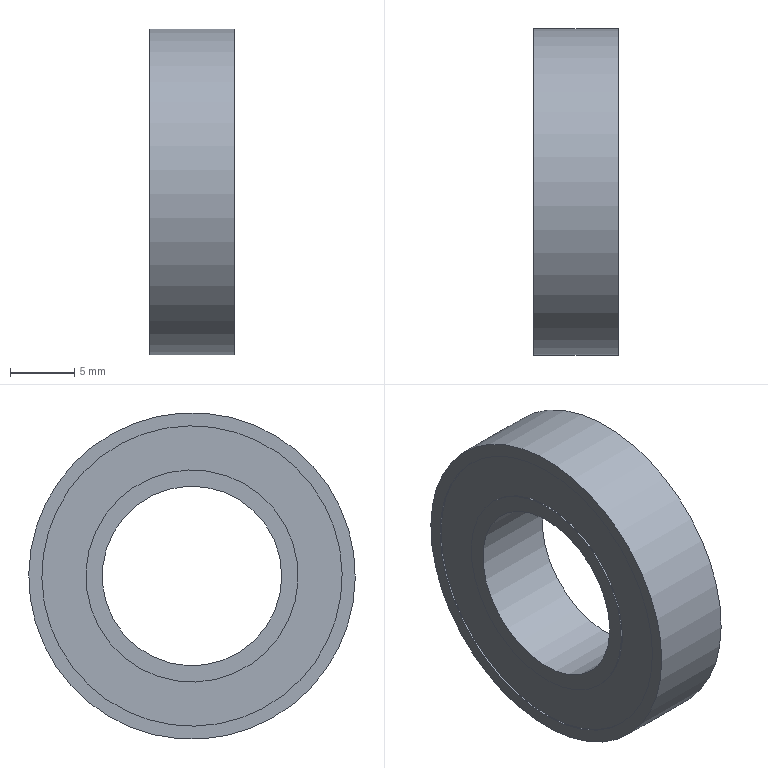Component | NX | BEARINGBIG | 3 solids | 12 faces | box 6.54 x 25.4 x 25.4 mm | volume 2257 mm3 | cylinder 6 | plane 6 | commonest cylinder face diameters 23.368 x2 16.51 x2 25.4 x1 13.97 x1
STEP:
#1=CARTESIAN_POINT('',(0.,0.,0.));
#2=DIRECTION('',(0.,0.,1.));
#3=DIRECTION('',(1.,0.,0.));
#4=AXIS2_PLACEMENT_3D('',#1,#2,#3);
#5=CARTESIAN_POINT('',(6.54,-10.403,-7.284));
#6=VERTEX_POINT('',#5);
#7=CARTESIAN_POINT('',(6.54,0.,0.));
#8=DIRECTION('',(1.,0.,0.));
#9=DIRECTION('',(0.,-0.8192,-0.5736));
#10=AXIS2_PLACEMENT_3D('',#7,#8,#9);
#11=CIRCLE('',#10,12.7);
#12=CARTESIAN_POINT('',(6.54,0.,0.));
#13=DIRECTION('',(-1.,0.,0.));
#14=DIRECTION('',(0.,0.5736,-0.8192));
#15=AXIS2_PLACEMENT_3D('',#12,#13,#14);
#16=CYLINDRICAL_SURFACE('',#15,12.7);
#17=CARTESIAN_POINT('',(7.854,0.));
#18=DIRECTION('',(-1.,0.));
#19=VECTOR('',#18,1.);
#20=LINE('',#17,#19);
#21=(GEOMETRIC_REPRESENTATION_CONTEXT(2)PARAMETRIC_REPRESENTATION_CONTEXT()REPRESENTATION_CONTEXT('',''));
#22=DEFINITIONAL_REPRESENTATION('',(#20),#21);
#23=PCURVE('',#16,#22);
#24=CARTESIAN_POINT('',(6.54,0.,0.));
#25=DIRECTION('',(1.,0.,0.));
#26=DIRECTION('',(0.,-0.5736,0.8192));
#27=AXIS2_PLACEMENT_3D('',#24,#25,#26);
#28=PLANE('',#27);
#29=CARTESIAN_POINT('',(0.,0.));
#30=DIRECTION('',(0.,1.));
#31=AXIS2_PLACEMENT_2D('',#29,#30);
#32=CIRCLE('',#31,12.7);
#33=(GEOMETRIC_REPRESENTATION_CONTEXT(2)PARAMETRIC_REPRESENTATION_CONTEXT()REPRESENTATION_CONTEXT('',''));
#34=DEFINITIONAL_REPRESENTATION('',(#32),#33);
#35=PCURVE('',#28,#34);
#36=SURFACE_CURVE('',#11,(#23,#35),.PCURVE_S1.);
#37=EDGE_CURVE('',#6,#6,#36,.T.);
#38=ORIENTED_EDGE('',*,*,#37,.F.);
#39=CARTESIAN_POINT('',(0.,-10.403,-7.284));
#40=VERTEX_POINT('',#39);
#41=CARTESIAN_POINT('',(6.54,-10.403,-7.284));
#42=CARTESIAN_POINT('',(0.,-10.403,-7.284));
#43=B_SPLINE_CURVE_WITH_KNOTS('',1,(#41,#42),.UNSPECIFIED.,.F.,.F.,(2,2),(0.,6.54),.PIECEWISE_BEZIER_KNOTS.);
#44=CARTESIAN_POINT('',(7.854,0.));
#45=DIRECTION('',(0.,1.));
#46=VECTOR('',#45,1.);
#47=LINE('',#44,#46);
#48=(GEOMETRIC_REPRESENTATION_CONTEXT(2)PARAMETRIC_REPRESENTATION_CONTEXT()REPRESENTATION_CONTEXT('',''));
#49=DEFINITIONAL_REPRESENTATION('',(#47),#48);
#50=PCURVE('',#16,#49);
#51=CARTESIAN_POINT('',(1.571,0.));
#52=DIRECTION('',(0.,1.));
#53=VECTOR('',#52,1.);
#54=LINE('',#51,#53);
#55=(GEOMETRIC_REPRESENTATION_CONTEXT(2)PARAMETRIC_REPRESENTATION_CONTEXT()REPRESENTATION_CONTEXT('',''));
#56=DEFINITIONAL_REPRESENTATION('',(#54),#55);
#57=PCURVE('',#16,#56);
#58=SEAM_CURVE('',#43,(#50,#57),.PCURVE_S1.);
#59=EDGE_CURVE('',#6,#40,#58,.T.);
#60=ORIENTED_EDGE('',*,*,#59,.T.);
#61=CARTESIAN_POINT('',(0.,0.,0.));
#62=DIRECTION('',(1.,0.,0.));
#63=DIRECTION('',(0.,-0.8192,-0.5736));
#64=AXIS2_PLACEMENT_3D('',#61,#62,#63);
#65=CIRCLE('',#64,12.7);
#66=CARTESIAN_POINT('',(7.854,6.54));
#67=DIRECTION('',(-1.,0.));
#68=VECTOR('',#67,1.);
#69=LINE('',#66,#68);
#70=(GEOMETRIC_REPRESENTATION_CONTEXT(2)PARAMETRIC_REPRESENTATION_CONTEXT()REPRESENTATION_CONTEXT('',''));
#71=DEFINITIONAL_REPRESENTATION('',(#69),#70);
#72=PCURVE('',#16,#71);
#73=CARTESIAN_POINT('',(0.,0.,0.));
#74=DIRECTION('',(1.,0.,0.));
#75=DIRECTION('',(0.,-0.5736,0.8192));
#76=AXIS2_PLACEMENT_3D('',#73,#74,#75);
#77=PLANE('',#76);
#78=CARTESIAN_POINT('',(0.,0.));
#79=DIRECTION('',(0.,1.));
#80=AXIS2_PLACEMENT_2D('',#78,#79);
#81=CIRCLE('',#80,12.7);
#82=(GEOMETRIC_REPRESENTATION_CONTEXT(2)PARAMETRIC_REPRESENTATION_CONTEXT()REPRESENTATION_CONTEXT('',''));
#83=DEFINITIONAL_REPRESENTATION('',(#81),#82);
#84=PCURVE('',#77,#83);
#85=SURFACE_CURVE('',#65,(#72,#84),.PCURVE_S1.);
#86=EDGE_CURVE('',#40,#40,#85,.T.);
#87=ORIENTED_EDGE('',*,*,#86,.T.);
#88=ORIENTED_EDGE('',*,*,#59,.F.);
#89=EDGE_LOOP('',(#38,#60,#87,#88));
#90=FACE_BOUND('',#89,.T.);
#91=ADVANCED_FACE('',(#90),#16,.T.);
#92=CARTESIAN_POINT('',(6.54,-9.571,-6.702));
#93=VERTEX_POINT('',#92);
#94=CARTESIAN_POINT('',(6.54,0.,0.));
#95=DIRECTION('',(-1.,0.,0.));
#96=DIRECTION('',(0.,-0.8192,-0.5736));
#97=AXIS2_PLACEMENT_3D('',#94,#95,#96);
#98=CIRCLE('',#97,11.684);
#99=CARTESIAN_POINT('',(6.54,0.,0.));
#100=DIRECTION('',(-1.,0.,0.));
#101=DIRECTION('',(0.,0.5736,-0.8192));
#102=AXIS2_PLACEMENT_3D('',#99,#100,#101);
#103=CYLINDRICAL_SURFACE('',#102,11.684);
#104=CARTESIAN_POINT('',(1.571,0.));
#105=DIRECTION('',(1.,0.));
#106=VECTOR('',#105,1.);
#107=LINE('',#104,#106);
#108=(GEOMETRIC_REPRESENTATION_CONTEXT(2)PARAMETRIC_REPRESENTATION_CONTEXT()REPRESENTATION_CONTEXT('',''));
#109=DEFINITIONAL_REPRESENTATION('',(#107),#108);
#110=PCURVE('',#103,#109);
#111=CARTESIAN_POINT('',(0.,11.684));
#112=CARTESIAN_POINT('',(20.237,11.684));
#113=CARTESIAN_POINT('',(10.119,-5.842));
#114=CARTESIAN_POINT('',(0.,-23.368));
#115=CARTESIAN_POINT('',(-10.119,-5.842));
#116=CARTESIAN_POINT('',(-20.237,11.684));
#117=CARTESIAN_POINT('',(0.,11.684));
#118=(BOUNDED_CURVE()B_SPLINE_CURVE(2,(#111,#112,#113,#114,#115,#116,#117),.UNSPECIFIED.,.T.,.F.)B_SPLINE_CURVE_WITH_KNOTS((1,2,2,2,2,1),(-2.094,0.,2.094,4.189,6.283,8.378),.UNSPECIFIED.)CURVE()GEOMETRIC_REPRESENTATION_ITEM()RATIONAL_B_SPLINE_CURVE((1.,0.5,1.,0.5,1.,0.5,1.))REPRESENTATION_ITEM(''));
#119=(GEOMETRIC_REPRESENTATION_CONTEXT(2)PARAMETRIC_REPRESENTATION_CONTEXT()REPRESENTATION_CONTEXT('',''));
#120=DEFINITIONAL_REPRESENTATION('',(#118),#119);
#121=PCURVE('',#28,#120);
#122=SURFACE_CURVE('',#98,(#110,#121),.PCURVE_S1.);
#123=EDGE_CURVE('',#93,#93,#122,.T.);
#124=ORIENTED_EDGE('',*,*,#123,.T.);
#125=CARTESIAN_POINT('',(0.,-9.571,-6.702));
#126=VERTEX_POINT('',#125);
#127=CARTESIAN_POINT('',(6.54,-9.571,-6.702));
#128=CARTESIAN_POINT('',(0.,-9.571,-6.702));
#129=B_SPLINE_CURVE_WITH_KNOTS('',1,(#127,#128),.UNSPECIFIED.,.F.,.F.,(2,2),(0.,6.54),.PIECEWISE_BEZIER_KNOTS.);
#130=CARTESIAN_POINT('',(7.854,0.));
#131=DIRECTION('',(0.,1.));
#132=VECTOR('',#131,1.);
#133=LINE('',#130,#132);
#134=(GEOMETRIC_REPRESENTATION_CONTEXT(2)PARAMETRIC_REPRESENTATION_CONTEXT()REPRESENTATION_CONTEXT('',''));
#135=DEFINITIONAL_REPRESENTATION('',(#133),#134);
#136=PCURVE('',#103,#135);
#137=CARTESIAN_POINT('',(1.571,0.));
#138=DIRECTION('',(0.,1.));
#139=VECTOR('',#138,1.);
#140=LINE('',#137,#139);
#141=(GEOMETRIC_REPRESENTATION_CONTEXT(2)PARAMETRIC_REPRESENTATION_CONTEXT()REPRESENTATION_CONTEXT('',''));
#142=DEFINITIONAL_REPRESENTATION('',(#140),#141);
#143=PCURVE('',#103,#142);
#144=SEAM_CURVE('',#129,(#136,#143),.PCURVE_S1.);
#145=EDGE_CURVE('',#93,#126,#144,.T.);
#146=ORIENTED_EDGE('',*,*,#145,.T.);
#147=CARTESIAN_POINT('',(0.,0.,0.));
#148=DIRECTION('',(-1.,0.,0.));
#149=DIRECTION('',(0.,-0.8192,-0.5736));
#150=AXIS2_PLACEMENT_3D('',#147,#148,#149);
#151=CIRCLE('',#150,11.684);
#152=CARTESIAN_POINT('',(1.571,6.54));
#153=DIRECTION('',(1.,0.));
#154=VECTOR('',#153,1.);
#155=LINE('',#152,#154);
#156=(GEOMETRIC_REPRESENTATION_CONTEXT(2)PARAMETRIC_REPRESENTATION_CONTEXT()REPRESENTATION_CONTEXT('',''));
#157=DEFINITIONAL_REPRESENTATION('',(#155),#156);
#158=PCURVE('',#103,#157);
#159=CARTESIAN_POINT('',(0.,11.684));
#160=CARTESIAN_POINT('',(20.237,11.684));
#161=CARTESIAN_POINT('',(10.119,-5.842));
#162=CARTESIAN_POINT('',(0.,-23.368));
#163=CARTESIAN_POINT('',(-10.119,-5.842));
#164=CARTESIAN_POINT('',(-20.237,11.684));
#165=CARTESIAN_POINT('',(0.,11.684));
#166=(BOUNDED_CURVE()B_SPLINE_CURVE(2,(#159,#160,#161,#162,#163,#164,#165),.UNSPECIFIED.,.T.,.F.)B_SPLINE_CURVE_WITH_KNOTS((1,2,2,2,2,1),(-2.094,0.,2.094,4.189,6.283,8.378),.UNSPECIFIED.)CURVE()GEOMETRIC_REPRESENTATION_ITEM()RATIONAL_B_SPLINE_CURVE((1.,0.5,1.,0.5,1.,0.5,1.))REPRESENTATION_ITEM(''));
#167=(GEOMETRIC_REPRESENTATION_CONTEXT(2)PARAMETRIC_REPRESENTATION_CONTEXT()REPRESENTATION_CONTEXT('',''));
#168=DEFINITIONAL_REPRESENTATION('',(#166),#167);
#169=PCURVE('',#77,#168);
#170=SURFACE_CURVE('',#151,(#158,#169),.PCURVE_S1.);
#171=EDGE_CURVE('',#126,#126,#170,.T.);
#172=ORIENTED_EDGE('',*,*,#171,.F.);
#173=ORIENTED_EDGE('',*,*,#145,.F.);
#174=EDGE_LOOP('',(#124,#146,#172,#173));
#175=FACE_BOUND('',#174,.F.);
#176=ADVANCED_FACE('',(#175),#103,.F.);
#177=ORIENTED_EDGE('',*,*,#37,.T.);
#178=EDGE_LOOP('',(#177));
#179=FACE_BOUND('',#178,.T.);
#180=ORIENTED_EDGE('',*,*,#123,.T.);
#181=EDGE_LOOP('',(#180));
#182=FACE_BOUND('',#181,.T.);
#183=ADVANCED_FACE('',(#179,#182),#28,.T.);
#184=ORIENTED_EDGE('',*,*,#86,.F.);
#185=EDGE_LOOP('',(#184));
#186=FACE_BOUND('',#185,.T.);
#187=ORIENTED_EDGE('',*,*,#171,.F.);
#188=EDGE_LOOP('',(#187));
#189=FACE_BOUND('',#188,.T.);
#190=ADVANCED_FACE('',(#186,#189),#77,.F.);
#191=CLOSED_SHELL('',(#91,#176,#183,#190));
#192=MANIFOLD_SOLID_BREP('',#191);
#193=(LENGTH_UNIT()NAMED_UNIT(*)SI_UNIT(.MILLI.,.METRE.));
#194=UNCERTAINTY_MEASURE_WITH_UNIT(LENGTH_MEASURE(0.00001),#193,'','');
#195=(NAMED_UNIT(*)PLANE_ANGLE_UNIT()SI_UNIT($,.RADIAN.));
#196=(NAMED_UNIT(*)SI_UNIT($,.STERADIAN.)SOLID_ANGLE_UNIT());
#197=(GEOMETRIC_REPRESENTATION_CONTEXT(3)GLOBAL_UNCERTAINTY_ASSIGNED_CONTEXT((#194))GLOBAL_UNIT_ASSIGNED_CONTEXT((#193,#195,#196))REPRESENTATION_CONTEXT('',''));
#198=ADVANCED_BREP_SHAPE_REPRESENTATION('',(#4,#192),#197);
#199=CARTESIAN_POINT('',(0.,0.,0.));
#200=DIRECTION('',(0.,0.,1.));
#201=DIRECTION('',(1.,0.,0.));
#202=AXIS2_PLACEMENT_3D('',#199,#200,#201);
#203=CARTESIAN_POINT('',(0.,0.,0.));
#204=DIRECTION('',(0.,0.,1.));
#205=DIRECTION('',(1.,0.,0.));
#206=AXIS2_PLACEMENT_3D('',#203,#204,#205);
#207=CARTESIAN_POINT('',(0.,0.,0.));
#208=DIRECTION('',(0.,0.,1.));
#209=DIRECTION('',(1.,0.,0.));
#210=AXIS2_PLACEMENT_3D('',#207,#208,#209);
#211=(LENGTH_UNIT()NAMED_UNIT(*)SI_UNIT(.MILLI.,.METRE.));
#212=UNCERTAINTY_MEASURE_WITH_UNIT(LENGTH_MEASURE(0.00001),#211,'','');
#213=(NAMED_UNIT(*)PLANE_ANGLE_UNIT()SI_UNIT($,.RADIAN.));
#214=(NAMED_UNIT(*)SI_UNIT($,.STERADIAN.)SOLID_ANGLE_UNIT());
#215=(GEOMETRIC_REPRESENTATION_CONTEXT(3)GLOBAL_UNCERTAINTY_ASSIGNED_CONTEXT((#212))GLOBAL_UNIT_ASSIGNED_CONTEXT((#211,#213,#214))REPRESENTATION_CONTEXT('',''));
#216=SHAPE_REPRESENTATION('',(#4,#202,#206,#210),#215);
#217=ITEM_DEFINED_TRANSFORMATION('','',#4,#202);
#218=(REPRESENTATION_RELATIONSHIP('','',#198,#216)REPRESENTATION_RELATIONSHIP_WITH_TRANSFORMATION(#217)SHAPE_REPRESENTATION_RELATIONSHIP());
#219=CARTESIAN_POINT('',(6.54,-6.762,-4.735));
#220=VERTEX_POINT('',#219);
#221=CARTESIAN_POINT('',(6.54,0.,0.));
#222=DIRECTION('',(-1.,0.,0.));
#223=DIRECTION('',(0.,-0.8192,-0.5736));
#224=AXIS2_PLACEMENT_3D('',#221,#222,#223);
#225=CIRCLE('',#224,8.255);
#226=CARTESIAN_POINT('',(6.54,0.,0.));
#227=DIRECTION('',(-1.,0.,0.));
#228=DIRECTION('',(0.,0.5736,-0.8192));
#229=AXIS2_PLACEMENT_3D('',#226,#227,#228);
#230=CYLINDRICAL_SURFACE('',#229,8.255);
#231=CARTESIAN_POINT('',(1.571,0.));
#232=DIRECTION('',(1.,0.));
#233=VECTOR('',#232,1.);
#234=LINE('',#231,#233);
#235=(GEOMETRIC_REPRESENTATION_CONTEXT(2)PARAMETRIC_REPRESENTATION_CONTEXT()REPRESENTATION_CONTEXT('',''));
#236=DEFINITIONAL_REPRESENTATION('',(#234),#235);
#237=PCURVE('',#230,#236);
#238=CARTESIAN_POINT('',(6.54,0.,0.));
#239=DIRECTION('',(1.,0.,0.));
#240=DIRECTION('',(0.,-0.5736,0.8192));
#241=AXIS2_PLACEMENT_3D('',#238,#239,#240);
#242=PLANE('',#241);
#243=CARTESIAN_POINT('',(0.,8.255));
#244=CARTESIAN_POINT('',(14.298,8.255));
#245=CARTESIAN_POINT('',(7.149,-4.128));
#246=CARTESIAN_POINT('',(0.,-16.51));
#247=CARTESIAN_POINT('',(-7.149,-4.128));
#248=CARTESIAN_POINT('',(-14.298,8.255));
#249=CARTESIAN_POINT('',(0.,8.255));
#250=(BOUNDED_CURVE()B_SPLINE_CURVE(2,(#243,#244,#245,#246,#247,#248,#249),.UNSPECIFIED.,.T.,.F.)B_SPLINE_CURVE_WITH_KNOTS((1,2,2,2,2,1),(-2.094,0.,2.094,4.189,6.283,8.378),.UNSPECIFIED.)CURVE()GEOMETRIC_REPRESENTATION_ITEM()RATIONAL_B_SPLINE_CURVE((1.,0.5,1.,0.5,1.,0.5,1.))REPRESENTATION_ITEM(''));
#251=(GEOMETRIC_REPRESENTATION_CONTEXT(2)PARAMETRIC_REPRESENTATION_CONTEXT()REPRESENTATION_CONTEXT('',''));
#252=DEFINITIONAL_REPRESENTATION('',(#250),#251);
#253=PCURVE('',#242,#252);
#254=SURFACE_CURVE('',#225,(#237,#253),.PCURVE_S1.);
#255=EDGE_CURVE('',#220,#220,#254,.T.);
#256=ORIENTED_EDGE('',*,*,#255,.T.);
#257=CARTESIAN_POINT('',(0.,-6.762,-4.735));
#258=VERTEX_POINT('',#257);
#259=CARTESIAN_POINT('',(6.54,-6.762,-4.735));
#260=CARTESIAN_POINT('',(0.,-6.762,-4.735));
#261=B_SPLINE_CURVE_WITH_KNOTS('',1,(#259,#260),.UNSPECIFIED.,.F.,.F.,(2,2),(0.,6.54),.PIECEWISE_BEZIER_KNOTS.);
#262=CARTESIAN_POINT('',(7.854,0.));
#263=DIRECTION('',(0.,1.));
#264=VECTOR('',#263,1.);
#265=LINE('',#262,#264);
#266=(GEOMETRIC_REPRESENTATION_CONTEXT(2)PARAMETRIC_REPRESENTATION_CONTEXT()REPRESENTATION_CONTEXT('',''));
#267=DEFINITIONAL_REPRESENTATION('',(#265),#266);
#268=PCURVE('',#230,#267);
#269=CARTESIAN_POINT('',(1.571,0.));
#270=DIRECTION('',(0.,1.));
#271=VECTOR('',#270,1.);
#272=LINE('',#269,#271);
#273=(GEOMETRIC_REPRESENTATION_CONTEXT(2)PARAMETRIC_REPRESENTATION_CONTEXT()REPRESENTATION_CONTEXT('',''));
#274=DEFINITIONAL_REPRESENTATION('',(#272),#273);
#275=PCURVE('',#230,#274);
#276=SEAM_CURVE('',#261,(#268,#275),.PCURVE_S1.);
#277=EDGE_CURVE('',#220,#258,#276,.T.);
#278=ORIENTED_EDGE('',*,*,#277,.T.);
#279=CARTESIAN_POINT('',(0.,0.,0.));
#280=DIRECTION('',(-1.,0.,0.));
#281=DIRECTION('',(0.,-0.8192,-0.5736));
#282=AXIS2_PLACEMENT_3D('',#279,#280,#281);
#283=CIRCLE('',#282,8.255);
#284=CARTESIAN_POINT('',(1.571,6.54));
#285=DIRECTION('',(1.,0.));
#286=VECTOR('',#285,1.);
#287=LINE('',#284,#286);
#288=(GEOMETRIC_REPRESENTATION_CONTEXT(2)PARAMETRIC_REPRESENTATION_CONTEXT()REPRESENTATION_CONTEXT('',''));
#289=DEFINITIONAL_REPRESENTATION('',(#287),#288);
#290=PCURVE('',#230,#289);
#291=CARTESIAN_POINT('',(0.,0.,0.));
#292=DIRECTION('',(1.,0.,0.));
#293=DIRECTION('',(0.,-0.5736,0.8192));
#294=AXIS2_PLACEMENT_3D('',#291,#292,#293);
#295=PLANE('',#294);
#296=CARTESIAN_POINT('',(0.,8.255));
#297=CARTESIAN_POINT('',(14.298,8.255));
#298=CARTESIAN_POINT('',(7.149,-4.128));
#299=CARTESIAN_POINT('',(0.,-16.51));
#300=CARTESIAN_POINT('',(-7.149,-4.128));
#301=CARTESIAN_POINT('',(-14.298,8.255));
#302=CARTESIAN_POINT('',(0.,8.255));
#303=(BOUNDED_CURVE()B_SPLINE_CURVE(2,(#296,#297,#298,#299,#300,#301,#302),.UNSPECIFIED.,.T.,.F.)B_SPLINE_CURVE_WITH_KNOTS((1,2,2,2,2,1),(-2.094,0.,2.094,4.189,6.283,8.378),.UNSPECIFIED.)CURVE()GEOMETRIC_REPRESENTATION_ITEM()RATIONAL_B_SPLINE_CURVE((1.,0.5,1.,0.5,1.,0.5,1.))REPRESENTATION_ITEM(''));
#304=(GEOMETRIC_REPRESENTATION_CONTEXT(2)PARAMETRIC_REPRESENTATION_CONTEXT()REPRESENTATION_CONTEXT('',''));
#305=DEFINITIONAL_REPRESENTATION('',(#303),#304);
#306=PCURVE('',#295,#305);
#307=SURFACE_CURVE('',#283,(#290,#306),.PCURVE_S1.);
#308=EDGE_CURVE('',#258,#258,#307,.T.);
#309=ORIENTED_EDGE('',*,*,#308,.F.);
#310=ORIENTED_EDGE('',*,*,#277,.F.);
#311=EDGE_LOOP('',(#256,#278,#309,#310));
#312=FACE_BOUND('',#311,.T.);
#313=ADVANCED_FACE('',(#312),#230,.T.);
#314=CARTESIAN_POINT('',(6.54,-5.722,-4.006));
#315=VERTEX_POINT('',#314);
#316=CARTESIAN_POINT('',(6.54,0.,0.));
#317=DIRECTION('',(1.,0.,0.));
#318=DIRECTION('',(0.,-0.8192,-0.5736));
#319=AXIS2_PLACEMENT_3D('',#316,#317,#318);
#320=CIRCLE('',#319,6.985);
#321=CARTESIAN_POINT('',(6.54,0.,0.));
#322=DIRECTION('',(-1.,0.,0.));
#323=DIRECTION('',(0.,0.5736,-0.8192));
#324=AXIS2_PLACEMENT_3D('',#321,#322,#323);
#325=CYLINDRICAL_SURFACE('',#324,6.985);
#326=CARTESIAN_POINT('',(7.854,0.));
#327=DIRECTION('',(-1.,0.));
#328=VECTOR('',#327,1.);
#329=LINE('',#326,#328);
#330=(GEOMETRIC_REPRESENTATION_CONTEXT(2)PARAMETRIC_REPRESENTATION_CONTEXT()REPRESENTATION_CONTEXT('',''));
#331=DEFINITIONAL_REPRESENTATION('',(#329),#330);
#332=PCURVE('',#325,#331);
#333=CARTESIAN_POINT('',(0.,0.));
#334=DIRECTION('',(0.,1.));
#335=AXIS2_PLACEMENT_2D('',#333,#334);
#336=CIRCLE('',#335,6.985);
#337=(GEOMETRIC_REPRESENTATION_CONTEXT(2)PARAMETRIC_REPRESENTATION_CONTEXT()REPRESENTATION_CONTEXT('',''));
#338=DEFINITIONAL_REPRESENTATION('',(#336),#337);
#339=PCURVE('',#242,#338);
#340=SURFACE_CURVE('',#320,(#332,#339),.PCURVE_S1.);
#341=EDGE_CURVE('',#315,#315,#340,.T.);
#342=ORIENTED_EDGE('',*,*,#341,.F.);
#343=CARTESIAN_POINT('',(0.,-5.722,-4.006));
#344=VERTEX_POINT('',#343);
#345=CARTESIAN_POINT('',(6.54,-5.722,-4.006));
#346=CARTESIAN_POINT('',(0.,-5.722,-4.006));
#347=B_SPLINE_CURVE_WITH_KNOTS('',1,(#345,#346),.UNSPECIFIED.,.F.,.F.,(2,2),(0.,6.54),.PIECEWISE_BEZIER_KNOTS.);
#348=CARTESIAN_POINT('',(7.854,0.));
#349=DIRECTION('',(0.,1.));
#350=VECTOR('',#349,1.);
#351=LINE('',#348,#350);
#352=(GEOMETRIC_REPRESENTATION_CONTEXT(2)PARAMETRIC_REPRESENTATION_CONTEXT()REPRESENTATION_CONTEXT('',''));
#353=DEFINITIONAL_REPRESENTATION('',(#351),#352);
#354=PCURVE('',#325,#353);
#355=CARTESIAN_POINT('',(1.571,0.));
#356=DIRECTION('',(0.,1.));
#357=VECTOR('',#356,1.);
#358=LINE('',#355,#357);
#359=(GEOMETRIC_REPRESENTATION_CONTEXT(2)PARAMETRIC_REPRESENTATION_CONTEXT()REPRESENTATION_CONTEXT('',''));
#360=DEFINITIONAL_REPRESENTATION('',(#358),#359);
#361=PCURVE('',#325,#360);
#362=SEAM_CURVE('',#347,(#354,#361),.PCURVE_S1.);
#363=EDGE_CURVE('',#315,#344,#362,.T.);
#364=ORIENTED_EDGE('',*,*,#363,.T.);
#365=CARTESIAN_POINT('',(0.,0.,0.));
#366=DIRECTION('',(1.,0.,0.));
#367=DIRECTION('',(0.,-0.8192,-0.5736));
#368=AXIS2_PLACEMENT_3D('',#365,#366,#367);
#369=CIRCLE('',#368,6.985);
#370=CARTESIAN_POINT('',(7.854,6.54));
#371=DIRECTION('',(-1.,0.));
#372=VECTOR('',#371,1.);
#373=LINE('',#370,#372);
#374=(GEOMETRIC_REPRESENTATION_CONTEXT(2)PARAMETRIC_REPRESENTATION_CONTEXT()REPRESENTATION_CONTEXT('',''));
#375=DEFINITIONAL_REPRESENTATION('',(#373),#374);
#376=PCURVE('',#325,#375);
#377=CARTESIAN_POINT('',(0.,0.));
#378=DIRECTION('',(0.,1.));
#379=AXIS2_PLACEMENT_2D('',#377,#378);
#380=CIRCLE('',#379,6.985);
#381=(GEOMETRIC_REPRESENTATION_CONTEXT(2)PARAMETRIC_REPRESENTATION_CONTEXT()REPRESENTATION_CONTEXT('',''));
#382=DEFINITIONAL_REPRESENTATION('',(#380),#381);
#383=PCURVE('',#295,#382);
#384=SURFACE_CURVE('',#369,(#376,#383),.PCURVE_S1.);
#385=EDGE_CURVE('',#344,#344,#384,.T.);
#386=ORIENTED_EDGE('',*,*,#385,.T.);
#387=ORIENTED_EDGE('',*,*,#363,.F.);
#388=EDGE_LOOP('',(#342,#364,#386,#387));
#389=FACE_BOUND('',#388,.F.);
#390=ADVANCED_FACE('',(#389),#325,.F.);
#391=ORIENTED_EDGE('',*,*,#255,.F.);
#392=EDGE_LOOP('',(#391));
#393=FACE_BOUND('',#392,.T.);
#394=ORIENTED_EDGE('',*,*,#341,.F.);
#395=EDGE_LOOP('',(#394));
#396=FACE_BOUND('',#395,.T.);
#397=ADVANCED_FACE('',(#393,#396),#242,.T.);
#398=ORIENTED_EDGE('',*,*,#308,.T.);
#399=EDGE_LOOP('',(#398));
#400=FACE_BOUND('',#399,.T.);
#401=ORIENTED_EDGE('',*,*,#385,.T.);
#402=EDGE_LOOP('',(#401));
#403=FACE_BOUND('',#402,.T.);
#404=ADVANCED_FACE('',(#400,#403),#295,.F.);
#405=CLOSED_SHELL('',(#313,#390,#397,#404));
#406=MANIFOLD_SOLID_BREP('',#405);
#407=(LENGTH_UNIT()NAMED_UNIT(*)SI_UNIT(.MILLI.,.METRE.));
#408=UNCERTAINTY_MEASURE_WITH_UNIT(LENGTH_MEASURE(0.00001),#407,'','');
#409=(NAMED_UNIT(*)PLANE_ANGLE_UNIT()SI_UNIT($,.RADIAN.));
#410=(NAMED_UNIT(*)SI_UNIT($,.STERADIAN.)SOLID_ANGLE_UNIT());
#411=(GEOMETRIC_REPRESENTATION_CONTEXT(3)GLOBAL_UNCERTAINTY_ASSIGNED_CONTEXT((#408))GLOBAL_UNIT_ASSIGNED_CONTEXT((#407,#409,#410))REPRESENTATION_CONTEXT('',''));
#412=ADVANCED_BREP_SHAPE_REPRESENTATION('',(#4,#406),#411);
#413=ITEM_DEFINED_TRANSFORMATION('','',#4,#206);
#414=(REPRESENTATION_RELATIONSHIP('','',#412,#216)REPRESENTATION_RELATIONSHIP_WITH_TRANSFORMATION(#413)SHAPE_REPRESENTATION_RELATIONSHIP());
#415=CARTESIAN_POINT('',(6.413,-9.571,-6.702));
#416=VERTEX_POINT('',#415);
#417=CARTESIAN_POINT('',(6.413,0.,0.));
#418=DIRECTION('',(1.,0.,0.));
#419=DIRECTION('',(0.,-0.8192,-0.5736));
#420=AXIS2_PLACEMENT_3D('',#417,#418,#419);
#421=CIRCLE('',#420,11.684);
#422=CARTESIAN_POINT('',(6.413,0.,0.));
#423=DIRECTION('',(-1.,0.,0.));
#424=DIRECTION('',(0.,0.5736,-0.8192));
#425=AXIS2_PLACEMENT_3D('',#422,#423,#424);
#426=CYLINDRICAL_SURFACE('',#425,11.684);
#427=CARTESIAN_POINT('',(7.854,0.));
#428=DIRECTION('',(-1.,0.));
#429=VECTOR('',#428,1.);
#430=LINE('',#427,#429);
#431=(GEOMETRIC_REPRESENTATION_CONTEXT(2)PARAMETRIC_REPRESENTATION_CONTEXT()REPRESENTATION_CONTEXT('',''));
#432=DEFINITIONAL_REPRESENTATION('',(#430),#431);
#433=PCURVE('',#426,#432);
#434=CARTESIAN_POINT('',(6.413,0.,0.));
#435=DIRECTION('',(1.,0.,0.));
#436=DIRECTION('',(0.,-0.5736,0.8192));
#437=AXIS2_PLACEMENT_3D('',#434,#435,#436);
#438=PLANE('',#437);
#439=CARTESIAN_POINT('',(0.,0.));
#440=DIRECTION('',(0.,1.));
#441=AXIS2_PLACEMENT_2D('',#439,#440);
#442=CIRCLE('',#441,11.684);
#443=(GEOMETRIC_REPRESENTATION_CONTEXT(2)PARAMETRIC_REPRESENTATION_CONTEXT()REPRESENTATION_CONTEXT('',''));
#444=DEFINITIONAL_REPRESENTATION('',(#442),#443);
#445=PCURVE('',#438,#444);
#446=SURFACE_CURVE('',#421,(#433,#445),.PCURVE_S1.);
#447=EDGE_CURVE('',#416,#416,#446,.T.);
#448=ORIENTED_EDGE('',*,*,#447,.F.);
#449=CARTESIAN_POINT('',(0.127,-9.571,-6.702));
#450=VERTEX_POINT('',#449);
#451=CARTESIAN_POINT('',(6.413,-9.571,-6.702));
#452=CARTESIAN_POINT('',(0.127,-9.571,-6.702));
#453=B_SPLINE_CURVE_WITH_KNOTS('',1,(#451,#452),.UNSPECIFIED.,.F.,.F.,(2,2),(0.,6.287),.PIECEWISE_BEZIER_KNOTS.);
#454=CARTESIAN_POINT('',(7.854,0.));
#455=DIRECTION('',(0.,1.));
#456=VECTOR('',#455,1.);
#457=LINE('',#454,#456);
#458=(GEOMETRIC_REPRESENTATION_CONTEXT(2)PARAMETRIC_REPRESENTATION_CONTEXT()REPRESENTATION_CONTEXT('',''));
#459=DEFINITIONAL_REPRESENTATION('',(#457),#458);
#460=PCURVE('',#426,#459);
#461=CARTESIAN_POINT('',(1.571,0.));
#462=DIRECTION('',(0.,1.));
#463=VECTOR('',#462,1.);
#464=LINE('',#461,#463);
#465=(GEOMETRIC_REPRESENTATION_CONTEXT(2)PARAMETRIC_REPRESENTATION_CONTEXT()REPRESENTATION_CONTEXT('',''));
#466=DEFINITIONAL_REPRESENTATION('',(#464),#465);
#467=PCURVE('',#426,#466);
#468=SEAM_CURVE('',#453,(#460,#467),.PCURVE_S1.);
#469=EDGE_CURVE('',#416,#450,#468,.T.);
#470=ORIENTED_EDGE('',*,*,#469,.T.);
#471=CARTESIAN_POINT('',(0.127,0.,0.));
#472=DIRECTION('',(1.,0.,0.));
#473=DIRECTION('',(0.,-0.8192,-0.5736));
#474=AXIS2_PLACEMENT_3D('',#471,#472,#473);
#475=CIRCLE('',#474,11.684);
#476=CARTESIAN_POINT('',(7.854,6.287));
#477=DIRECTION('',(-1.,0.));
#478=VECTOR('',#477,1.);
#479=LINE('',#476,#478);
#480=(GEOMETRIC_REPRESENTATION_CONTEXT(2)PARAMETRIC_REPRESENTATION_CONTEXT()REPRESENTATION_CONTEXT('',''));
#481=DEFINITIONAL_REPRESENTATION('',(#479),#480);
#482=PCURVE('',#426,#481);
#483=CARTESIAN_POINT('',(0.127,0.,0.));
#484=DIRECTION('',(1.,0.,0.));
#485=DIRECTION('',(0.,-0.5736,0.8192));
#486=AXIS2_PLACEMENT_3D('',#483,#484,#485);
#487=PLANE('',#486);
#488=CARTESIAN_POINT('',(0.,0.));
#489=DIRECTION('',(0.,1.));
#490=AXIS2_PLACEMENT_2D('',#488,#489);
#491=CIRCLE('',#490,11.684);
#492=(GEOMETRIC_REPRESENTATION_CONTEXT(2)PARAMETRIC_REPRESENTATION_CONTEXT()REPRESENTATION_CONTEXT('',''));
#493=DEFINITIONAL_REPRESENTATION('',(#491),#492);
#494=PCURVE('',#487,#493);
#495=SURFACE_CURVE('',#475,(#482,#494),.PCURVE_S1.);
#496=EDGE_CURVE('',#450,#450,#495,.T.);
#497=ORIENTED_EDGE('',*,*,#496,.T.);
#498=ORIENTED_EDGE('',*,*,#469,.F.);
#499=EDGE_LOOP('',(#448,#470,#497,#498));
#500=FACE_BOUND('',#499,.T.);
#501=ADVANCED_FACE('',(#500),#426,.T.);
#502=CARTESIAN_POINT('',(6.413,-6.762,-4.735));
#503=VERTEX_POINT('',#502);
#504=CARTESIAN_POINT('',(6.413,0.,0.));
#505=DIRECTION('',(1.,0.,0.));
#506=DIRECTION('',(0.,-0.8192,-0.5736));
#507=AXIS2_PLACEMENT_3D('',#504,#505,#506);
#508=CIRCLE('',#507,8.255);
#509=CARTESIAN_POINT('',(6.413,0.,0.));
#510=DIRECTION('',(-1.,0.,0.));
#511=DIRECTION('',(0.,0.5736,-0.8192));
#512=AXIS2_PLACEMENT_3D('',#509,#510,#511);
#513=CYLINDRICAL_SURFACE('',#512,8.255);
#514=CARTESIAN_POINT('',(7.854,0.));
#515=DIRECTION('',(-1.,0.));
#516=VECTOR('',#515,1.);
#517=LINE('',#514,#516);
#518=(GEOMETRIC_REPRESENTATION_CONTEXT(2)PARAMETRIC_REPRESENTATION_CONTEXT()REPRESENTATION_CONTEXT('',''));
#519=DEFINITIONAL_REPRESENTATION('',(#517),#518);
#520=PCURVE('',#513,#519);
#521=CARTESIAN_POINT('',(0.,0.));
#522=DIRECTION('',(0.,1.));
#523=AXIS2_PLACEMENT_2D('',#521,#522);
#524=CIRCLE('',#523,8.255);
#525=(GEOMETRIC_REPRESENTATION_CONTEXT(2)PARAMETRIC_REPRESENTATION_CONTEXT()REPRESENTATION_CONTEXT('',''));
#526=DEFINITIONAL_REPRESENTATION('',(#524),#525);
#527=PCURVE('',#438,#526);
#528=SURFACE_CURVE('',#508,(#520,#527),.PCURVE_S1.);
#529=EDGE_CURVE('',#503,#503,#528,.T.);
#530=ORIENTED_EDGE('',*,*,#529,.F.);
#531=CARTESIAN_POINT('',(0.127,-6.762,-4.735));
#532=VERTEX_POINT('',#531);
#533=CARTESIAN_POINT('',(6.413,-6.762,-4.735));
#534=CARTESIAN_POINT('',(0.127,-6.762,-4.735));
#535=B_SPLINE_CURVE_WITH_KNOTS('',1,(#533,#534),.UNSPECIFIED.,.F.,.F.,(2,2),(0.,6.287),.PIECEWISE_BEZIER_KNOTS.);
#536=CARTESIAN_POINT('',(7.854,0.));
#537=DIRECTION('',(0.,1.));
#538=VECTOR('',#537,1.);
#539=LINE('',#536,#538);
#540=(GEOMETRIC_REPRESENTATION_CONTEXT(2)PARAMETRIC_REPRESENTATION_CONTEXT()REPRESENTATION_CONTEXT('',''));
#541=DEFINITIONAL_REPRESENTATION('',(#539),#540);
#542=PCURVE('',#513,#541);
#543=CARTESIAN_POINT('',(1.571,0.));
#544=DIRECTION('',(0.,1.));
#545=VECTOR('',#544,1.);
#546=LINE('',#543,#545);
#547=(GEOMETRIC_REPRESENTATION_CONTEXT(2)PARAMETRIC_REPRESENTATION_CONTEXT()REPRESENTATION_CONTEXT('',''));
#548=DEFINITIONAL_REPRESENTATION('',(#546),#547);
#549=PCURVE('',#513,#548);
#550=SEAM_CURVE('',#535,(#542,#549),.PCURVE_S1.);
#551=EDGE_CURVE('',#503,#532,#550,.T.);
#552=ORIENTED_EDGE('',*,*,#551,.T.);
#553=CARTESIAN_POINT('',(0.127,0.,0.));
#554=DIRECTION('',(1.,0.,0.));
#555=DIRECTION('',(0.,-0.8192,-0.5736));
#556=AXIS2_PLACEMENT_3D('',#553,#554,#555);
#557=CIRCLE('',#556,8.255);
#558=CARTESIAN_POINT('',(7.854,6.287));
#559=DIRECTION('',(-1.,0.));
#560=VECTOR('',#559,1.);
#561=LINE('',#558,#560);
#562=(GEOMETRIC_REPRESENTATION_CONTEXT(2)PARAMETRIC_REPRESENTATION_CONTEXT()REPRESENTATION_CONTEXT('',''));
#563=DEFINITIONAL_REPRESENTATION('',(#561),#562);
#564=PCURVE('',#513,#563);
#565=CARTESIAN_POINT('',(0.,0.));
#566=DIRECTION('',(0.,1.));
#567=AXIS2_PLACEMENT_2D('',#565,#566);
#568=CIRCLE('',#567,8.255);
#569=(GEOMETRIC_REPRESENTATION_CONTEXT(2)PARAMETRIC_REPRESENTATION_CONTEXT()REPRESENTATION_CONTEXT('',''));
#570=DEFINITIONAL_REPRESENTATION('',(#568),#569);
#571=PCURVE('',#487,#570);
#572=SURFACE_CURVE('',#557,(#564,#571),.PCURVE_S1.);
#573=EDGE_CURVE('',#532,#532,#572,.T.);
#574=ORIENTED_EDGE('',*,*,#573,.T.);
#575=ORIENTED_EDGE('',*,*,#551,.F.);
#576=EDGE_LOOP('',(#530,#552,#574,#575));
#577=FACE_BOUND('',#576,.F.);
#578=ADVANCED_FACE('',(#577),#513,.F.);
#579=ORIENTED_EDGE('',*,*,#447,.T.);
#580=EDGE_LOOP('',(#579));
#581=FACE_BOUND('',#580,.T.);
#582=ORIENTED_EDGE('',*,*,#529,.F.);
#583=EDGE_LOOP('',(#582));
#584=FACE_BOUND('',#583,.T.);
#585=ADVANCED_FACE('',(#581,#584),#438,.T.);
#586=ORIENTED_EDGE('',*,*,#496,.F.);
#587=EDGE_LOOP('',(#586));
#588=FACE_BOUND('',#587,.T.);
#589=ORIENTED_EDGE('',*,*,#573,.T.);
#590=EDGE_LOOP('',(#589));
#591=FACE_BOUND('',#590,.T.);
#592=ADVANCED_FACE('',(#588,#591),#487,.F.);
#593=CLOSED_SHELL('',(#501,#578,#585,#592));
#594=MANIFOLD_SOLID_BREP('',#593);
#595=(LENGTH_UNIT()NAMED_UNIT(*)SI_UNIT(.MILLI.,.METRE.));
#596=UNCERTAINTY_MEASURE_WITH_UNIT(LENGTH_MEASURE(0.00001),#595,'','');
#597=(NAMED_UNIT(*)PLANE_ANGLE_UNIT()SI_UNIT($,.RADIAN.));
#598=(NAMED_UNIT(*)SI_UNIT($,.STERADIAN.)SOLID_ANGLE_UNIT());
#599=(GEOMETRIC_REPRESENTATION_CONTEXT(3)GLOBAL_UNCERTAINTY_ASSIGNED_CONTEXT((#596))GLOBAL_UNIT_ASSIGNED_CONTEXT((#595,#597,#598))REPRESENTATION_CONTEXT('',''));
#600=ADVANCED_BREP_SHAPE_REPRESENTATION('',(#4,#594),#599);
#601=ITEM_DEFINED_TRANSFORMATION('','',#4,#210);
#602=(REPRESENTATION_RELATIONSHIP('','',#600,#216)REPRESENTATION_RELATIONSHIP_WITH_TRANSFORMATION(#601)SHAPE_REPRESENTATION_RELATIONSHIP());